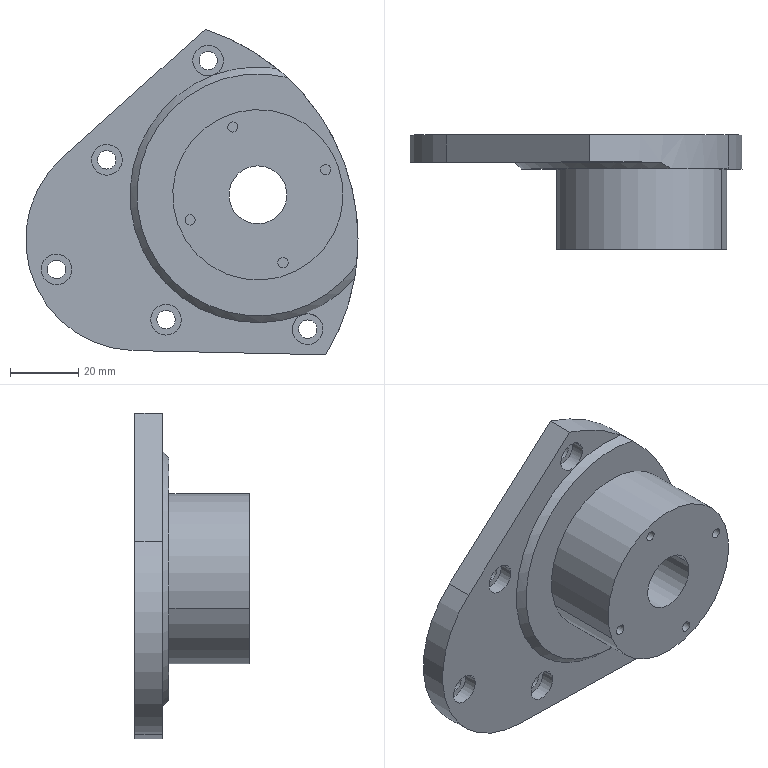Component | SolidWorks | Gear cover festo-1 | 1 solid | 76 faces | box 97.5 x 33.5 x 95.51 mm | volume 88034 mm3 | cylinder 39 | plane 22 | cone 14 | torus 1 | commonest cylinder face diameters 9 x10 5.4 x10 3 x8 50 x2 17 x2 130 x2 52 x2 4 x2